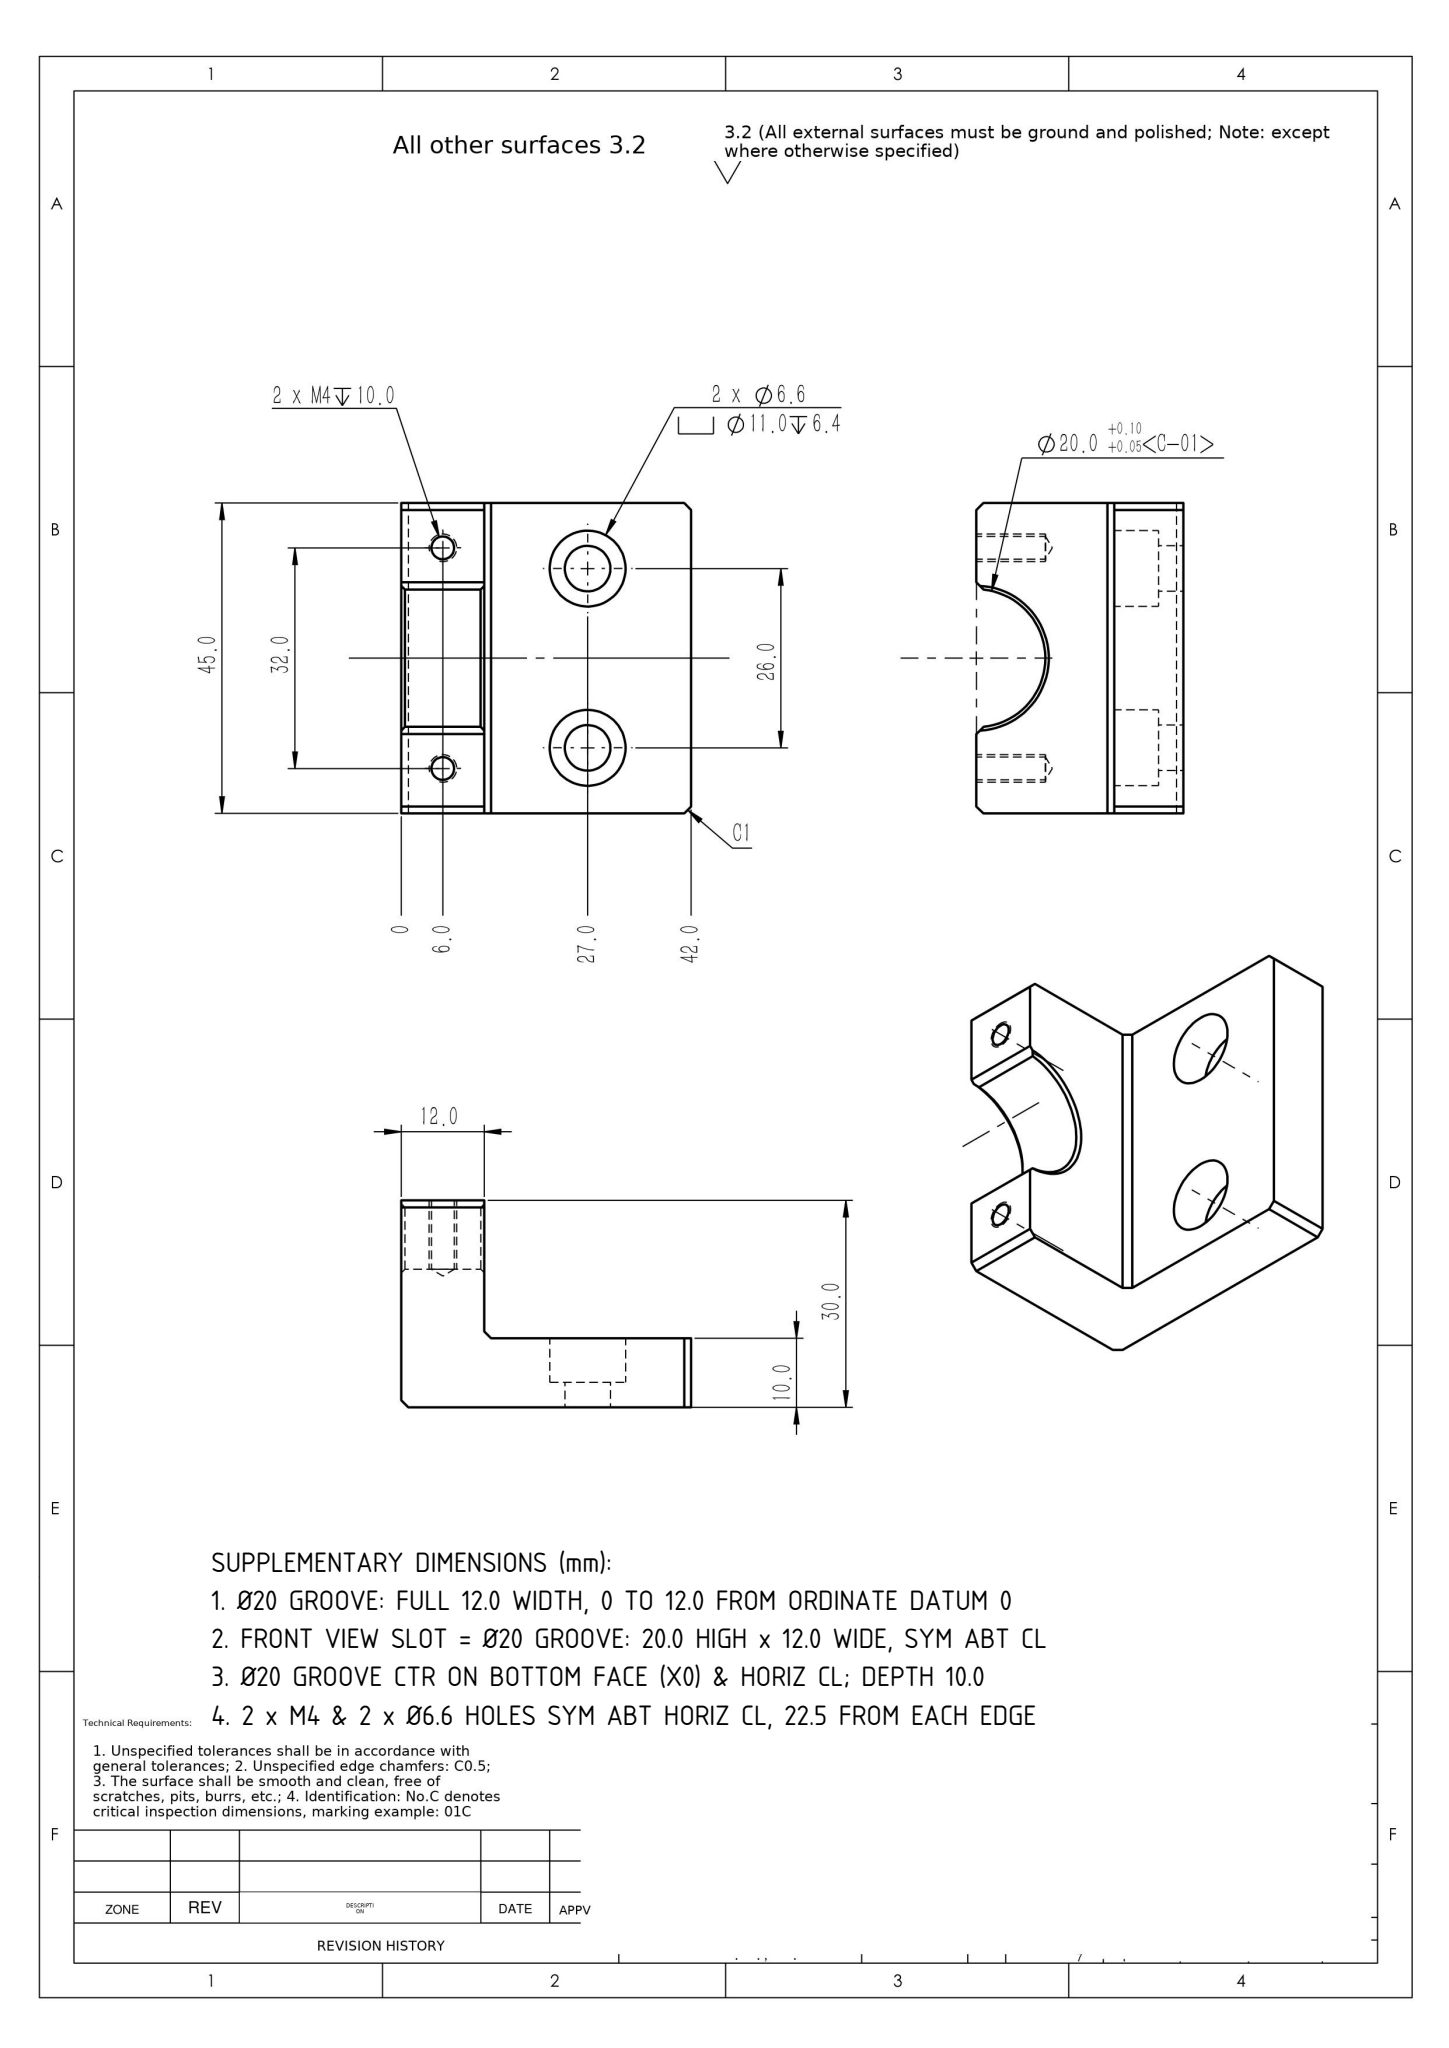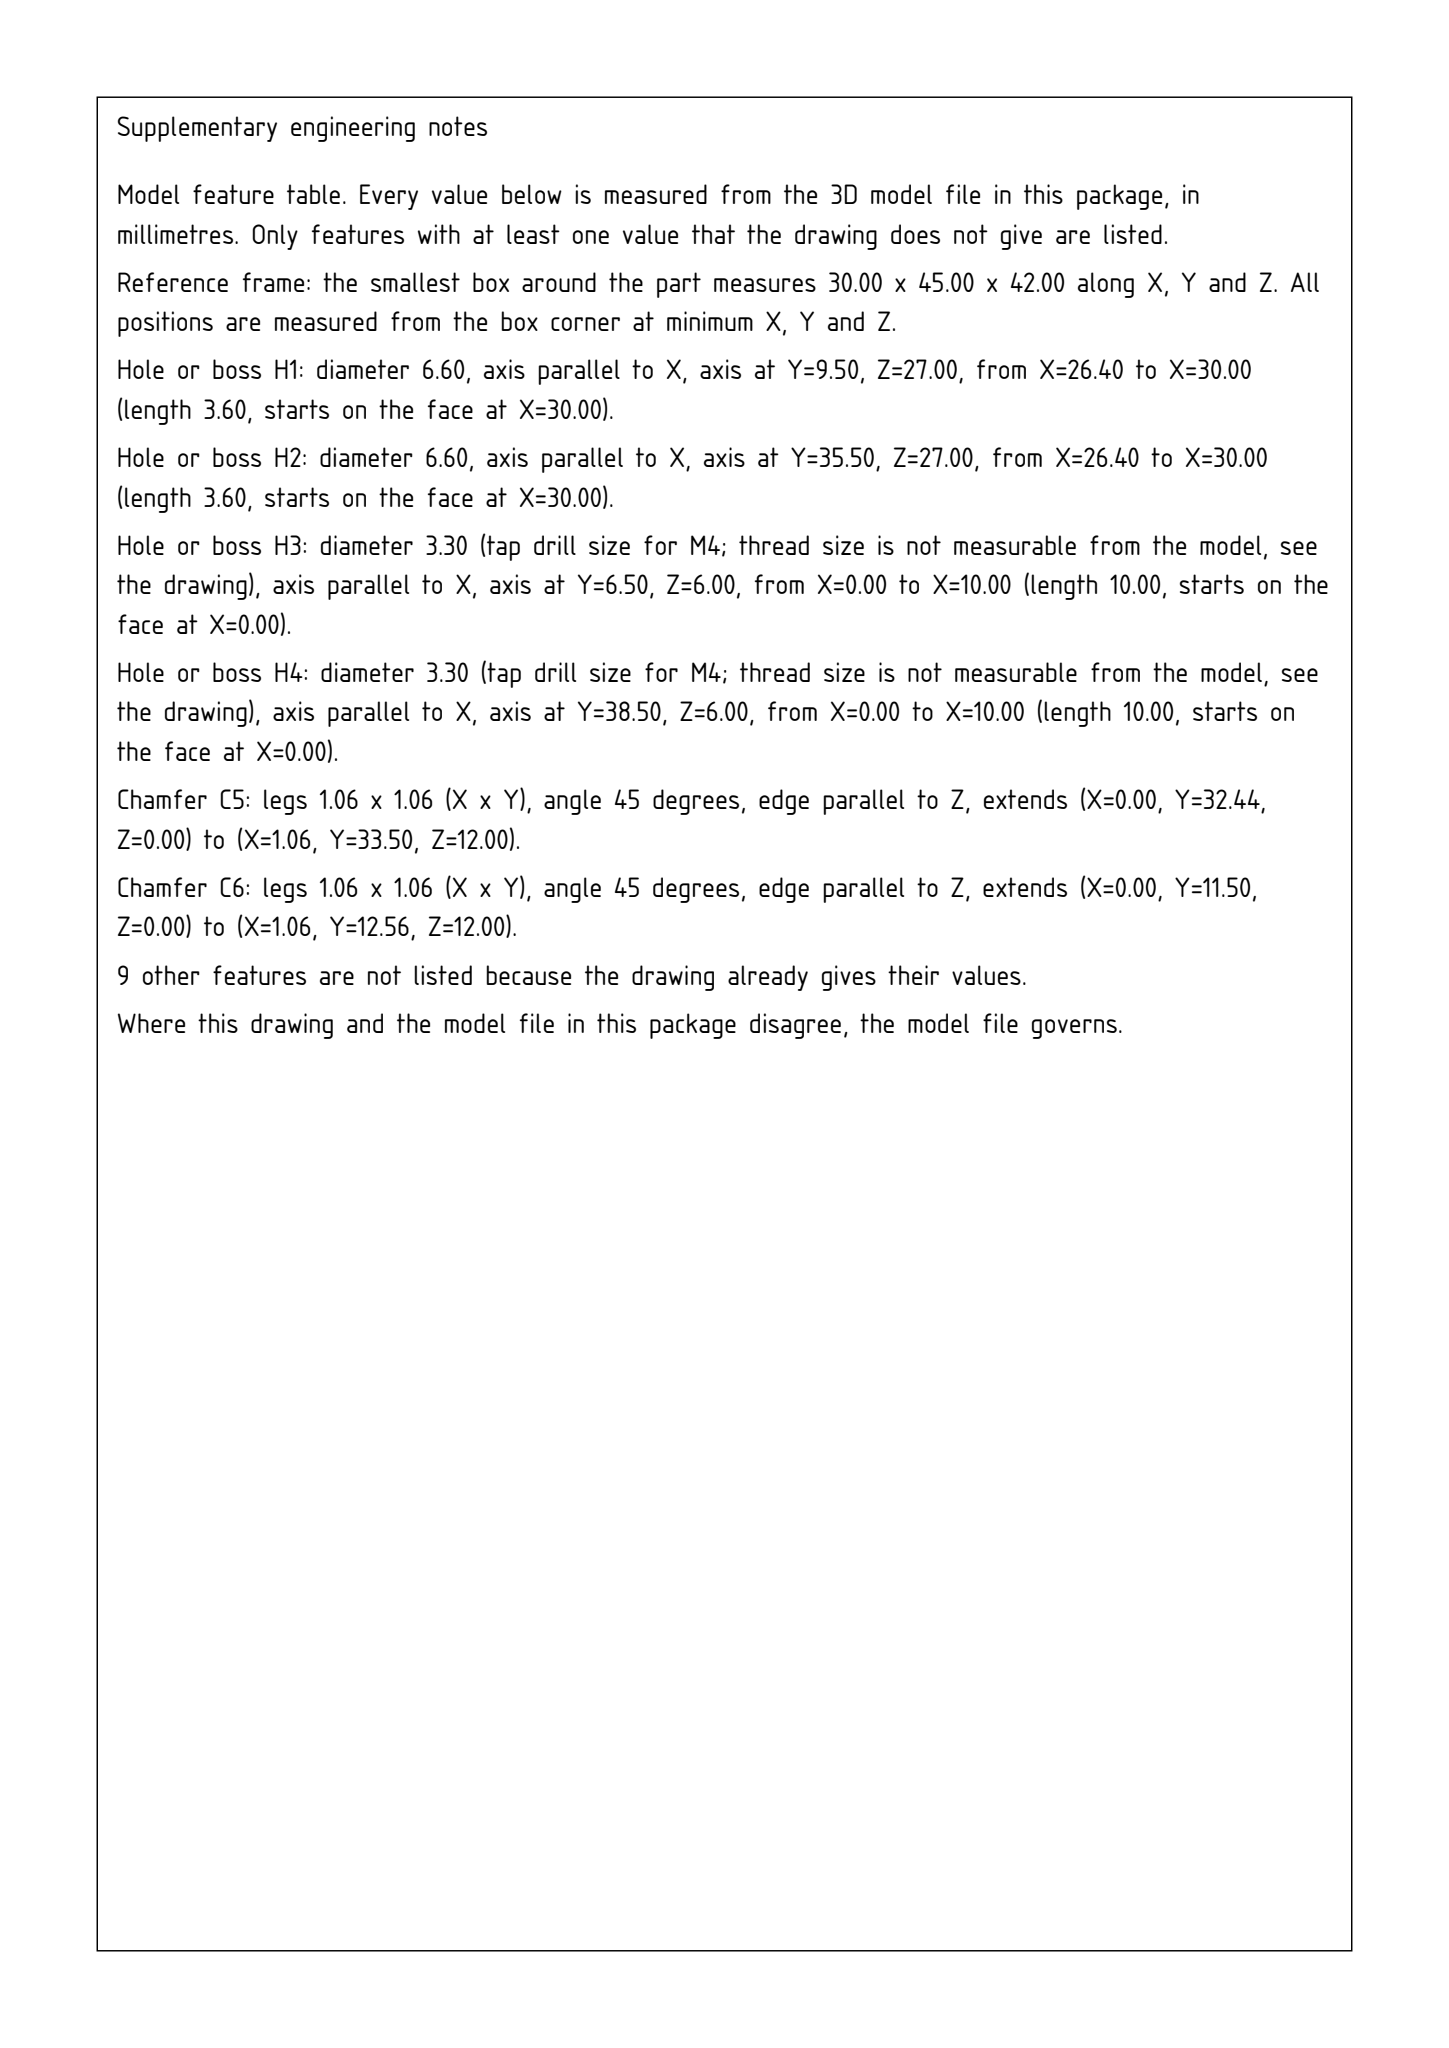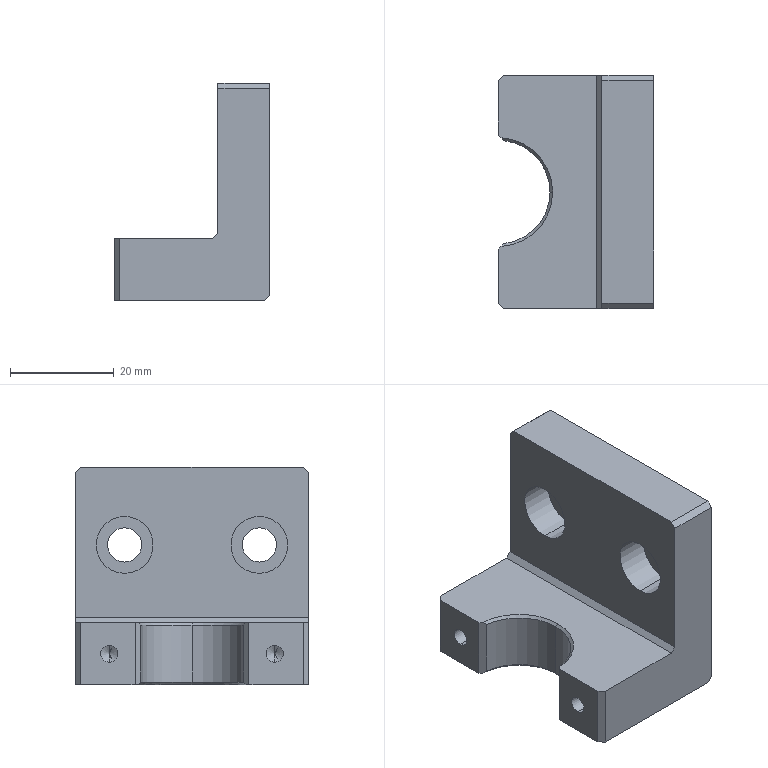Part | SolidWorks | mm | 1 solid | 40 faces | box 30 x 45 x 42 mm | volume 26134 mm3 | plane 19 | cylinder 14 | cone 7 | commonest cylinder face diameters 3.3 x4 11 x4 6.6 x4 20 x2